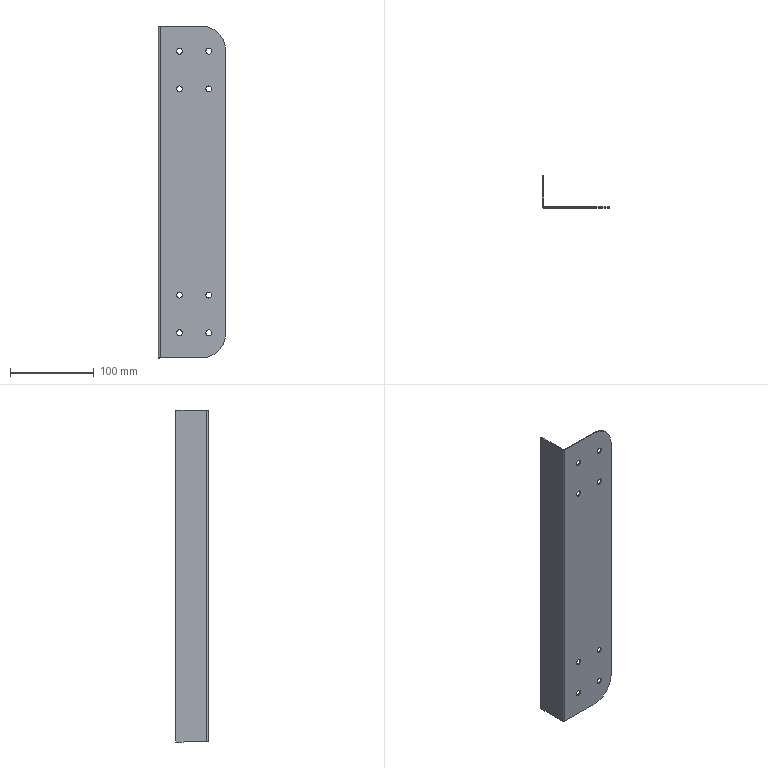Component | SolidWorks | dbj3-1_w13-1 | 1 solid | 32 faces | box 80 x 38.5 x 396 mm | volume 68176 mm3 | cylinder 20 | plane 12 | commonest cylinder face diameters 7 x16 58 x2 4 x1 1 x1
STEP:
#1=COLOUR_RGB('',0.7922,0.8196,0.9333);
#2=FILL_AREA_STYLE_COLOUR('',#1);
#3=FILL_AREA_STYLE('',(#2));
#4=SURFACE_STYLE_FILL_AREA(#3);
#5=SURFACE_SIDE_STYLE('',(#4));
#6=SURFACE_STYLE_USAGE(.BOTH.,#5);
#7=PRESENTATION_STYLE_ASSIGNMENT((#6));
#8=CARTESIAN_POINT('',(8.996,-31.014,8.445));
#9=VERTEX_POINT('',#8);
#10=CARTESIAN_POINT('',(8.996,-31.014,8.72));
#11=VERTEX_POINT('',#10);
#12=CARTESIAN_POINT('',(8.996,-31.014,8.583));
#13=DIRECTION('',(0.,-1.,0.));
#14=DIRECTION('',(0.,0.,1.));
#15=AXIS2_PLACEMENT_3D('',#12,#13,#14);
#16=CIRCLE('',#15,0.1378);
#17=EDGE_CURVE('',#9,#11,#16,.T.);
#18=ORIENTED_EDGE('',*,*,#17,.F.);
#19=CARTESIAN_POINT('',(8.996,-31.073,8.445));
#20=VERTEX_POINT('',#19);
#21=CARTESIAN_POINT('',(8.996,-30.679,8.445));
#22=DIRECTION('',(0.,-1.,0.));
#23=VECTOR('',#22,39.37);
#24=LINE('',#21,#23);
#25=EDGE_CURVE('',#9,#20,#24,.T.);
#26=ORIENTED_EDGE('',*,*,#25,.T.);
#27=CARTESIAN_POINT('',(8.996,-31.073,8.72));
#28=VERTEX_POINT('',#27);
#29=CARTESIAN_POINT('',(8.996,-31.073,8.583));
#30=DIRECTION('',(0.,-1.,0.));
#31=DIRECTION('',(0.,0.,-1.));
#32=AXIS2_PLACEMENT_3D('',#29,#30,#31);
#33=CIRCLE('',#32,0.1378);
#34=EDGE_CURVE('',#20,#28,#33,.T.);
#35=ORIENTED_EDGE('',*,*,#34,.T.);
#36=CARTESIAN_POINT('',(8.996,-30.679,8.72));
#37=DIRECTION('',(0.,-1.,0.));
#38=VECTOR('',#37,39.37);
#39=LINE('',#36,#38);
#40=EDGE_CURVE('',#11,#28,#39,.T.);
#41=ORIENTED_EDGE('',*,*,#40,.F.);
#42=EDGE_LOOP('',(#18,#26,#35,#41));
#43=FACE_OUTER_BOUND('',#42,.T.);
#44=CARTESIAN_POINT('',(8.996,-30.679,8.583));
#45=DIRECTION('',(0.,-1.,0.));
#46=DIRECTION('',(0.,0.,1.));
#47=AXIS2_PLACEMENT_3D('',#44,#45,#46);
#48=CYLINDRICAL_SURFACE('',#47,0.1378);
#49=ADVANCED_FACE('',(#43),#48,.F.);
#50=CARTESIAN_POINT('',(7.618,-31.014,8.445));
#51=VERTEX_POINT('',#50);
#52=CARTESIAN_POINT('',(7.618,-31.014,8.72));
#53=VERTEX_POINT('',#52);
#54=CARTESIAN_POINT('',(7.618,-31.014,8.583));
#55=DIRECTION('',(0.,-1.,0.));
#56=DIRECTION('',(0.,0.,1.));
#57=AXIS2_PLACEMENT_3D('',#54,#55,#56);
#58=CIRCLE('',#57,0.1378);
#59=EDGE_CURVE('',#51,#53,#58,.T.);
#60=ORIENTED_EDGE('',*,*,#59,.F.);
#61=CARTESIAN_POINT('',(7.618,-31.073,8.445));
#62=VERTEX_POINT('',#61);
#63=CARTESIAN_POINT('',(7.618,-30.679,8.445));
#64=DIRECTION('',(0.,-1.,0.));
#65=VECTOR('',#64,39.37);
#66=LINE('',#63,#65);
#67=EDGE_CURVE('',#51,#62,#66,.T.);
#68=ORIENTED_EDGE('',*,*,#67,.T.);
#69=CARTESIAN_POINT('',(7.618,-31.073,8.72));
#70=VERTEX_POINT('',#69);
#71=CARTESIAN_POINT('',(7.618,-31.073,8.583));
#72=DIRECTION('',(0.,-1.,0.));
#73=DIRECTION('',(0.,0.,-1.));
#74=AXIS2_PLACEMENT_3D('',#71,#72,#73);
#75=CIRCLE('',#74,0.1378);
#76=EDGE_CURVE('',#62,#70,#75,.T.);
#77=ORIENTED_EDGE('',*,*,#76,.T.);
#78=CARTESIAN_POINT('',(7.618,-30.679,8.72));
#79=DIRECTION('',(0.,-1.,0.));
#80=VECTOR('',#79,39.37);
#81=LINE('',#78,#80);
#82=EDGE_CURVE('',#53,#70,#81,.T.);
#83=ORIENTED_EDGE('',*,*,#82,.F.);
#84=EDGE_LOOP('',(#60,#68,#77,#83));
#85=FACE_OUTER_BOUND('',#84,.T.);
#86=CARTESIAN_POINT('',(7.618,-30.679,8.583));
#87=DIRECTION('',(0.,-1.,0.));
#88=DIRECTION('',(0.,0.,1.));
#89=AXIS2_PLACEMENT_3D('',#86,#87,#88);
#90=CYLINDRICAL_SURFACE('',#89,0.1378);
#91=ADVANCED_FACE('',(#85),#90,.F.);
#92=CARTESIAN_POINT('',(7.618,-31.014,6.673));
#93=VERTEX_POINT('',#92);
#94=CARTESIAN_POINT('',(7.618,-31.014,6.949));
#95=VERTEX_POINT('',#94);
#96=CARTESIAN_POINT('',(7.618,-31.014,6.811));
#97=DIRECTION('',(0.,-1.,0.));
#98=DIRECTION('',(0.,0.,1.));
#99=AXIS2_PLACEMENT_3D('',#96,#97,#98);
#100=CIRCLE('',#99,0.1378);
#101=EDGE_CURVE('',#93,#95,#100,.T.);
#102=ORIENTED_EDGE('',*,*,#101,.F.);
#103=CARTESIAN_POINT('',(7.618,-31.073,6.673));
#104=VERTEX_POINT('',#103);
#105=CARTESIAN_POINT('',(7.618,-30.679,6.673));
#106=DIRECTION('',(0.,-1.,0.));
#107=VECTOR('',#106,39.37);
#108=LINE('',#105,#107);
#109=EDGE_CURVE('',#93,#104,#108,.T.);
#110=ORIENTED_EDGE('',*,*,#109,.T.);
#111=CARTESIAN_POINT('',(7.618,-31.073,6.949));
#112=VERTEX_POINT('',#111);
#113=CARTESIAN_POINT('',(7.618,-31.073,6.811));
#114=DIRECTION('',(0.,-1.,0.));
#115=DIRECTION('',(0.,0.,-1.));
#116=AXIS2_PLACEMENT_3D('',#113,#114,#115);
#117=CIRCLE('',#116,0.1378);
#118=EDGE_CURVE('',#104,#112,#117,.T.);
#119=ORIENTED_EDGE('',*,*,#118,.T.);
#120=CARTESIAN_POINT('',(7.618,-30.679,6.949));
#121=DIRECTION('',(0.,-1.,0.));
#122=VECTOR('',#121,39.37);
#123=LINE('',#120,#122);
#124=EDGE_CURVE('',#95,#112,#123,.T.);
#125=ORIENTED_EDGE('',*,*,#124,.F.);
#126=EDGE_LOOP('',(#102,#110,#119,#125));
#127=FACE_OUTER_BOUND('',#126,.T.);
#128=CARTESIAN_POINT('',(7.618,-30.679,6.811));
#129=DIRECTION('',(0.,-1.,0.));
#130=DIRECTION('',(0.,0.,1.));
#131=AXIS2_PLACEMENT_3D('',#128,#129,#130);
#132=CYLINDRICAL_SURFACE('',#131,0.1378);
#133=ADVANCED_FACE('',(#127),#132,.F.);
#134=CARTESIAN_POINT('',(8.996,-31.014,6.673));
#135=VERTEX_POINT('',#134);
#136=CARTESIAN_POINT('',(8.996,-31.014,6.949));
#137=VERTEX_POINT('',#136);
#138=CARTESIAN_POINT('',(8.996,-31.014,6.811));
#139=DIRECTION('',(0.,-1.,0.));
#140=DIRECTION('',(0.,0.,1.));
#141=AXIS2_PLACEMENT_3D('',#138,#139,#140);
#142=CIRCLE('',#141,0.1378);
#143=EDGE_CURVE('',#135,#137,#142,.T.);
#144=ORIENTED_EDGE('',*,*,#143,.F.);
#145=CARTESIAN_POINT('',(8.996,-31.073,6.673));
#146=VERTEX_POINT('',#145);
#147=CARTESIAN_POINT('',(8.996,-30.679,6.673));
#148=DIRECTION('',(0.,-1.,0.));
#149=VECTOR('',#148,39.37);
#150=LINE('',#147,#149);
#151=EDGE_CURVE('',#135,#146,#150,.T.);
#152=ORIENTED_EDGE('',*,*,#151,.T.);
#153=CARTESIAN_POINT('',(8.996,-31.073,6.949));
#154=VERTEX_POINT('',#153);
#155=CARTESIAN_POINT('',(8.996,-31.073,6.811));
#156=DIRECTION('',(0.,-1.,0.));
#157=DIRECTION('',(0.,0.,-1.));
#158=AXIS2_PLACEMENT_3D('',#155,#156,#157);
#159=CIRCLE('',#158,0.1378);
#160=EDGE_CURVE('',#146,#154,#159,.T.);
#161=ORIENTED_EDGE('',*,*,#160,.T.);
#162=CARTESIAN_POINT('',(8.996,-30.679,6.949));
#163=DIRECTION('',(0.,-1.,0.));
#164=VECTOR('',#163,39.37);
#165=LINE('',#162,#164);
#166=EDGE_CURVE('',#137,#154,#165,.T.);
#167=ORIENTED_EDGE('',*,*,#166,.F.);
#168=EDGE_LOOP('',(#144,#152,#161,#167));
#169=FACE_OUTER_BOUND('',#168,.T.);
#170=CARTESIAN_POINT('',(8.996,-30.679,6.811));
#171=DIRECTION('',(0.,-1.,0.));
#172=DIRECTION('',(0.,0.,1.));
#173=AXIS2_PLACEMENT_3D('',#170,#171,#172);
#174=CYLINDRICAL_SURFACE('',#173,0.1378);
#175=ADVANCED_FACE('',(#169),#174,.F.);
#176=CARTESIAN_POINT('',(8.996,-31.014,-3.012));
#177=VERTEX_POINT('',#176);
#178=CARTESIAN_POINT('',(8.996,-31.014,-2.736));
#179=VERTEX_POINT('',#178);
#180=CARTESIAN_POINT('',(8.996,-31.014,-2.874));
#181=DIRECTION('',(0.,-1.,0.));
#182=DIRECTION('',(0.,0.,1.));
#183=AXIS2_PLACEMENT_3D('',#180,#181,#182);
#184=CIRCLE('',#183,0.1378);
#185=EDGE_CURVE('',#177,#179,#184,.T.);
#186=ORIENTED_EDGE('',*,*,#185,.F.);
#187=CARTESIAN_POINT('',(8.996,-31.073,-3.012));
#188=VERTEX_POINT('',#187);
#189=CARTESIAN_POINT('',(8.996,-30.679,-3.012));
#190=DIRECTION('',(0.,-1.,0.));
#191=VECTOR('',#190,39.37);
#192=LINE('',#189,#191);
#193=EDGE_CURVE('',#177,#188,#192,.T.);
#194=ORIENTED_EDGE('',*,*,#193,.T.);
#195=CARTESIAN_POINT('',(8.996,-31.073,-2.736));
#196=VERTEX_POINT('',#195);
#197=CARTESIAN_POINT('',(8.996,-31.073,-2.874));
#198=DIRECTION('',(0.,-1.,0.));
#199=DIRECTION('',(0.,0.,1.));
#200=AXIS2_PLACEMENT_3D('',#197,#198,#199);
#201=CIRCLE('',#200,0.1378);
#202=EDGE_CURVE('',#188,#196,#201,.T.);
#203=ORIENTED_EDGE('',*,*,#202,.T.);
#204=CARTESIAN_POINT('',(8.996,-30.679,-2.736));
#205=DIRECTION('',(0.,-1.,0.));
#206=VECTOR('',#205,39.37);
#207=LINE('',#204,#206);
#208=EDGE_CURVE('',#179,#196,#207,.T.);
#209=ORIENTED_EDGE('',*,*,#208,.F.);
#210=EDGE_LOOP('',(#186,#194,#203,#209));
#211=FACE_OUTER_BOUND('',#210,.T.);
#212=CARTESIAN_POINT('',(8.996,-30.679,-2.874));
#213=DIRECTION('',(0.,-1.,0.));
#214=DIRECTION('',(0.,0.,1.));
#215=AXIS2_PLACEMENT_3D('',#212,#213,#214);
#216=CYLINDRICAL_SURFACE('',#215,0.1378);
#217=ADVANCED_FACE('',(#211),#216,.F.);
#218=CARTESIAN_POINT('',(7.618,-31.014,-3.012));
#219=VERTEX_POINT('',#218);
#220=CARTESIAN_POINT('',(7.618,-31.014,-2.736));
#221=VERTEX_POINT('',#220);
#222=CARTESIAN_POINT('',(7.618,-31.014,-2.874));
#223=DIRECTION('',(0.,-1.,0.));
#224=DIRECTION('',(0.,0.,1.));
#225=AXIS2_PLACEMENT_3D('',#222,#223,#224);
#226=CIRCLE('',#225,0.1378);
#227=EDGE_CURVE('',#219,#221,#226,.T.);
#228=ORIENTED_EDGE('',*,*,#227,.F.);
#229=CARTESIAN_POINT('',(7.618,-31.073,-3.012));
#230=VERTEX_POINT('',#229);
#231=CARTESIAN_POINT('',(7.618,-30.679,-3.012));
#232=DIRECTION('',(0.,-1.,0.));
#233=VECTOR('',#232,39.37);
#234=LINE('',#231,#233);
#235=EDGE_CURVE('',#219,#230,#234,.T.);
#236=ORIENTED_EDGE('',*,*,#235,.T.);
#237=CARTESIAN_POINT('',(7.618,-31.073,-2.736));
#238=VERTEX_POINT('',#237);
#239=CARTESIAN_POINT('',(7.618,-31.073,-2.874));
#240=DIRECTION('',(0.,-1.,0.));
#241=DIRECTION('',(0.,0.,1.));
#242=AXIS2_PLACEMENT_3D('',#239,#240,#241);
#243=CIRCLE('',#242,0.1378);
#244=EDGE_CURVE('',#230,#238,#243,.T.);
#245=ORIENTED_EDGE('',*,*,#244,.T.);
#246=CARTESIAN_POINT('',(7.618,-30.679,-2.736));
#247=DIRECTION('',(0.,-1.,0.));
#248=VECTOR('',#247,39.37);
#249=LINE('',#246,#248);
#250=EDGE_CURVE('',#221,#238,#249,.T.);
#251=ORIENTED_EDGE('',*,*,#250,.F.);
#252=EDGE_LOOP('',(#228,#236,#245,#251));
#253=FACE_OUTER_BOUND('',#252,.T.);
#254=CARTESIAN_POINT('',(7.618,-30.679,-2.874));
#255=DIRECTION('',(0.,-1.,0.));
#256=DIRECTION('',(0.,0.,1.));
#257=AXIS2_PLACEMENT_3D('',#254,#255,#256);
#258=CYLINDRICAL_SURFACE('',#257,0.1378);
#259=ADVANCED_FACE('',(#253),#258,.F.);
#260=CARTESIAN_POINT('',(7.618,-31.014,-4.783));
#261=VERTEX_POINT('',#260);
#262=CARTESIAN_POINT('',(7.618,-31.014,-4.508));
#263=VERTEX_POINT('',#262);
#264=CARTESIAN_POINT('',(7.618,-31.014,-4.646));
#265=DIRECTION('',(0.,-1.,0.));
#266=DIRECTION('',(0.,0.,1.));
#267=AXIS2_PLACEMENT_3D('',#264,#265,#266);
#268=CIRCLE('',#267,0.1378);
#269=EDGE_CURVE('',#261,#263,#268,.T.);
#270=ORIENTED_EDGE('',*,*,#269,.F.);
#271=CARTESIAN_POINT('',(7.618,-31.073,-4.783));
#272=VERTEX_POINT('',#271);
#273=CARTESIAN_POINT('',(7.618,-30.679,-4.783));
#274=DIRECTION('',(0.,-1.,0.));
#275=VECTOR('',#274,39.37);
#276=LINE('',#273,#275);
#277=EDGE_CURVE('',#261,#272,#276,.T.);
#278=ORIENTED_EDGE('',*,*,#277,.T.);
#279=CARTESIAN_POINT('',(7.618,-31.073,-4.508));
#280=VERTEX_POINT('',#279);
#281=CARTESIAN_POINT('',(7.618,-31.073,-4.646));
#282=DIRECTION('',(0.,-1.,0.));
#283=DIRECTION('',(0.,0.,1.));
#284=AXIS2_PLACEMENT_3D('',#281,#282,#283);
#285=CIRCLE('',#284,0.1378);
#286=EDGE_CURVE('',#272,#280,#285,.T.);
#287=ORIENTED_EDGE('',*,*,#286,.T.);
#288=CARTESIAN_POINT('',(7.618,-30.679,-4.508));
#289=DIRECTION('',(0.,-1.,0.));
#290=VECTOR('',#289,39.37);
#291=LINE('',#288,#290);
#292=EDGE_CURVE('',#263,#280,#291,.T.);
#293=ORIENTED_EDGE('',*,*,#292,.F.);
#294=EDGE_LOOP('',(#270,#278,#287,#293));
#295=FACE_OUTER_BOUND('',#294,.T.);
#296=CARTESIAN_POINT('',(7.618,-30.679,-4.646));
#297=DIRECTION('',(0.,-1.,0.));
#298=DIRECTION('',(0.,0.,1.));
#299=AXIS2_PLACEMENT_3D('',#296,#297,#298);
#300=CYLINDRICAL_SURFACE('',#299,0.1378);
#301=ADVANCED_FACE('',(#295),#300,.F.);
#302=CARTESIAN_POINT('',(8.996,-31.014,-4.783));
#303=VERTEX_POINT('',#302);
#304=CARTESIAN_POINT('',(8.996,-31.014,-4.508));
#305=VERTEX_POINT('',#304);
#306=CARTESIAN_POINT('',(8.996,-31.014,-4.646));
#307=DIRECTION('',(0.,-1.,0.));
#308=DIRECTION('',(0.,0.,1.));
#309=AXIS2_PLACEMENT_3D('',#306,#307,#308);
#310=CIRCLE('',#309,0.1378);
#311=EDGE_CURVE('',#303,#305,#310,.T.);
#312=ORIENTED_EDGE('',*,*,#311,.F.);
#313=CARTESIAN_POINT('',(8.996,-31.073,-4.783));
#314=VERTEX_POINT('',#313);
#315=CARTESIAN_POINT('',(8.996,-30.679,-4.783));
#316=DIRECTION('',(0.,-1.,0.));
#317=VECTOR('',#316,39.37);
#318=LINE('',#315,#317);
#319=EDGE_CURVE('',#303,#314,#318,.T.);
#320=ORIENTED_EDGE('',*,*,#319,.T.);
#321=CARTESIAN_POINT('',(8.996,-31.073,-4.508));
#322=VERTEX_POINT('',#321);
#323=CARTESIAN_POINT('',(8.996,-31.073,-4.646));
#324=DIRECTION('',(0.,-1.,0.));
#325=DIRECTION('',(0.,0.,1.));
#326=AXIS2_PLACEMENT_3D('',#323,#324,#325);
#327=CIRCLE('',#326,0.1378);
#328=EDGE_CURVE('',#314,#322,#327,.T.);
#329=ORIENTED_EDGE('',*,*,#328,.T.);
#330=CARTESIAN_POINT('',(8.996,-30.679,-4.508));
#331=DIRECTION('',(0.,-1.,0.));
#332=VECTOR('',#331,39.37);
#333=LINE('',#330,#332);
#334=EDGE_CURVE('',#305,#322,#333,.T.);
#335=ORIENTED_EDGE('',*,*,#334,.F.);
#336=EDGE_LOOP('',(#312,#320,#329,#335));
#337=FACE_OUTER_BOUND('',#336,.T.);
#338=CARTESIAN_POINT('',(8.996,-30.679,-4.646));
#339=DIRECTION('',(0.,-1.,0.));
#340=DIRECTION('',(0.,0.,1.));
#341=AXIS2_PLACEMENT_3D('',#338,#339,#340);
#342=CYLINDRICAL_SURFACE('',#341,0.1378);
#343=ADVANCED_FACE('',(#337),#342,.F.);
#344=CARTESIAN_POINT('',(6.634,-30.994,9.764));
#345=VERTEX_POINT('',#344);
#346=CARTESIAN_POINT('',(6.693,-30.994,9.764));
#347=VERTEX_POINT('',#346);
#348=CARTESIAN_POINT('',(6.634,-30.994,9.764));
#349=DIRECTION('',(1.,0.,-0.));
#350=VECTOR('',#349,39.37);
#351=LINE('',#348,#350);
#352=EDGE_CURVE('',#345,#347,#351,.T.);
#353=ORIENTED_EDGE('',*,*,#352,.F.);
#354=CARTESIAN_POINT('',(6.713,-31.073,9.764));
#355=VERTEX_POINT('',#354);
#356=CARTESIAN_POINT('',(6.713,-30.994,9.764));
#357=DIRECTION('',(-0.,-0.,-1.));
#358=DIRECTION('',(-1.,0.,0.));
#359=AXIS2_PLACEMENT_3D('',#356,#357,#358);
#360=CIRCLE('',#359,0.07874);
#361=EDGE_CURVE('',#355,#345,#360,.T.);
#362=ORIENTED_EDGE('',*,*,#361,.F.);
#363=CARTESIAN_POINT('',(6.713,-31.014,9.764));
#364=VERTEX_POINT('',#363);
#365=CARTESIAN_POINT('',(6.713,-31.014,9.764));
#366=DIRECTION('',(0.,-1.,0.));
#367=VECTOR('',#366,39.37);
#368=LINE('',#365,#367);
#369=EDGE_CURVE('',#364,#355,#368,.T.);
#370=ORIENTED_EDGE('',*,*,#369,.F.);
#371=CARTESIAN_POINT('',(6.713,-30.994,9.764));
#372=DIRECTION('',(-0.,-0.,-1.));
#373=DIRECTION('',(-1.,0.,0.));
#374=AXIS2_PLACEMENT_3D('',#371,#372,#373);
#375=CIRCLE('',#374,0.01969);
#376=EDGE_CURVE('',#364,#347,#375,.T.);
#377=ORIENTED_EDGE('',*,*,#376,.T.);
#378=EDGE_LOOP('',(#353,#362,#370,#377));
#379=FACE_OUTER_BOUND('',#378,.T.);
#380=CARTESIAN_POINT('',(6.634,-30.994,9.764));
#381=DIRECTION('',(0.,0.,1.));
#382=DIRECTION('',(-1.,-0.,0.));
#383=AXIS2_PLACEMENT_3D('',#380,#381,#382);
#384=PLANE('',#383);
#385=ADVANCED_FACE('',(#379),#384,.T.);
#386=CARTESIAN_POINT('',(6.634,-29.557,9.764));
#387=VERTEX_POINT('',#386);
#388=CARTESIAN_POINT('',(6.634,-31.073,9.764));
#389=DIRECTION('',(-0.,1.,-0.));
#390=VECTOR('',#389,39.37);
#391=LINE('',#388,#390);
#392=EDGE_CURVE('',#345,#387,#391,.T.);
#393=ORIENTED_EDGE('',*,*,#392,.F.);
#394=ORIENTED_EDGE('',*,*,#352,.T.);
#395=CARTESIAN_POINT('',(6.693,-29.557,9.764));
#396=VERTEX_POINT('',#395);
#397=CARTESIAN_POINT('',(6.693,-31.073,9.764));
#398=DIRECTION('',(-0.,1.,-0.));
#399=VECTOR('',#398,39.37);
#400=LINE('',#397,#399);
#401=EDGE_CURVE('',#347,#396,#400,.T.);
#402=ORIENTED_EDGE('',*,*,#401,.T.);
#403=CARTESIAN_POINT('',(6.634,-29.557,9.764));
#404=DIRECTION('',(1.,0.,-0.));
#405=VECTOR('',#404,39.37);
#406=LINE('',#403,#405);
#407=EDGE_CURVE('',#387,#396,#406,.T.);
#408=ORIENTED_EDGE('',*,*,#407,.F.);
#409=EDGE_LOOP('',(#393,#394,#402,#408));
#410=FACE_OUTER_BOUND('',#409,.T.);
#411=CARTESIAN_POINT('',(6.713,-31.014,9.764));
#412=DIRECTION('',(0.,0.,1.));
#413=DIRECTION('',(-1.,-0.,0.));
#414=AXIS2_PLACEMENT_3D('',#411,#412,#413);
#415=PLANE('',#414);
#416=ADVANCED_FACE('',(#410),#415,.T.);
#417=CARTESIAN_POINT('',(6.713,-31.073,-5.827));
#418=VERTEX_POINT('',#417);
#419=CARTESIAN_POINT('',(6.713,-31.014,-5.827));
#420=VERTEX_POINT('',#419);
#421=CARTESIAN_POINT('',(6.713,-31.073,-5.827));
#422=DIRECTION('',(-0.,1.,-0.));
#423=VECTOR('',#422,39.37);
#424=LINE('',#421,#423);
#425=EDGE_CURVE('',#418,#420,#424,.T.);
#426=ORIENTED_EDGE('',*,*,#425,.F.);
#427=CARTESIAN_POINT('',(6.634,-30.994,-5.827));
#428=VERTEX_POINT('',#427);
#429=CARTESIAN_POINT('',(6.713,-30.994,-5.827));
#430=DIRECTION('',(-0.,-0.,-1.));
#431=DIRECTION('',(-1.,0.,0.));
#432=AXIS2_PLACEMENT_3D('',#429,#430,#431);
#433=CIRCLE('',#432,0.07874);
#434=EDGE_CURVE('',#418,#428,#433,.T.);
#435=ORIENTED_EDGE('',*,*,#434,.T.);
#436=CARTESIAN_POINT('',(6.693,-30.994,-5.827));
#437=VERTEX_POINT('',#436);
#438=CARTESIAN_POINT('',(6.693,-30.994,-5.827));
#439=DIRECTION('',(-1.,-0.,0.));
#440=VECTOR('',#439,39.37);
#441=LINE('',#438,#440);
#442=EDGE_CURVE('',#437,#428,#441,.T.);
#443=ORIENTED_EDGE('',*,*,#442,.F.);
#444=CARTESIAN_POINT('',(6.713,-30.994,-5.827));
#445=DIRECTION('',(-0.,-0.,-1.));
#446=DIRECTION('',(-1.,0.,0.));
#447=AXIS2_PLACEMENT_3D('',#444,#445,#446);
#448=CIRCLE('',#447,0.01969);
#449=EDGE_CURVE('',#420,#437,#448,.T.);
#450=ORIENTED_EDGE('',*,*,#449,.F.);
#451=EDGE_LOOP('',(#426,#435,#443,#450));
#452=FACE_OUTER_BOUND('',#451,.T.);
#453=CARTESIAN_POINT('',(6.713,-31.073,-5.827));
#454=DIRECTION('',(-0.,-0.,-1.));
#455=DIRECTION('',(1.,0.,-0.));
#456=AXIS2_PLACEMENT_3D('',#453,#454,#455);
#457=PLANE('',#456);
#458=ADVANCED_FACE('',(#452),#457,.T.);
#459=CARTESIAN_POINT('',(8.642,-31.014,-5.827));
#460=VERTEX_POINT('',#459);
#461=CARTESIAN_POINT('',(9.783,-31.014,-5.827));
#462=DIRECTION('',(-1.,-0.,0.));
#463=VECTOR('',#462,39.37);
#464=LINE('',#461,#463);
#465=EDGE_CURVE('',#460,#420,#464,.T.);
#466=ORIENTED_EDGE('',*,*,#465,.F.);
#467=CARTESIAN_POINT('',(8.642,-31.073,-5.827));
#468=VERTEX_POINT('',#467);
#469=CARTESIAN_POINT('',(8.642,-30.994,-5.827));
#470=DIRECTION('',(0.,-1.,0.));
#471=VECTOR('',#470,39.37);
#472=LINE('',#469,#471);
#473=EDGE_CURVE('',#460,#468,#472,.T.);
#474=ORIENTED_EDGE('',*,*,#473,.T.);
#475=CARTESIAN_POINT('',(9.783,-31.073,-5.827));
#476=DIRECTION('',(-1.,-0.,0.));
#477=VECTOR('',#476,39.37);
#478=LINE('',#475,#477);
#479=EDGE_CURVE('',#468,#418,#478,.T.);
#480=ORIENTED_EDGE('',*,*,#479,.T.);
#481=ORIENTED_EDGE('',*,*,#425,.T.);
#482=EDGE_LOOP('',(#466,#474,#480,#481));
#483=FACE_OUTER_BOUND('',#482,.T.);
#484=CARTESIAN_POINT('',(6.693,-30.994,-5.827));
#485=DIRECTION('',(-0.,-0.,-1.));
#486=DIRECTION('',(1.,0.,-0.));
#487=AXIS2_PLACEMENT_3D('',#484,#485,#486);
#488=PLANE('',#487);
#489=ADVANCED_FACE('',(#483),#488,.T.);
#490=CARTESIAN_POINT('',(6.693,-29.557,-5.827));
#491=VERTEX_POINT('',#490);
#492=CARTESIAN_POINT('',(6.693,-31.073,-5.827));
#493=DIRECTION('',(-0.,1.,-0.));
#494=VECTOR('',#493,39.37);
#495=LINE('',#492,#494);
#496=EDGE_CURVE('',#437,#491,#495,.T.);
#497=ORIENTED_EDGE('',*,*,#496,.T.);
#498=CARTESIAN_POINT('',(6.693,-29.557,9.764));
#499=DIRECTION('',(-0.,-0.,-1.));
#500=VECTOR('',#499,39.37);
#501=LINE('',#498,#500);
#502=EDGE_CURVE('',#396,#491,#501,.T.);
#503=ORIENTED_EDGE('',*,*,#502,.F.);
#504=ORIENTED_EDGE('',*,*,#401,.F.);
#505=CARTESIAN_POINT('',(6.693,-30.994,9.764));
#506=DIRECTION('',(-0.,-0.,-1.));
#507=VECTOR('',#506,39.37);
#508=LINE('',#505,#507);
#509=EDGE_CURVE('',#347,#437,#508,.T.);
#510=ORIENTED_EDGE('',*,*,#509,.T.);
#511=EDGE_LOOP('',(#497,#503,#504,#510));
#512=FACE_OUTER_BOUND('',#511,.T.);
#513=CARTESIAN_POINT('',(6.693,-31.073,9.764));
#514=DIRECTION('',(-1.,-0.,0.));
#515=DIRECTION('',(0.,-1.,0.));
#516=AXIS2_PLACEMENT_3D('',#513,#514,#515);
#517=PLANE('',#516);
#518=ADVANCED_FACE('',(#512),#517,.F.);
#519=CARTESIAN_POINT('',(6.634,-29.557,-5.827));
#520=VERTEX_POINT('',#519);
#521=CARTESIAN_POINT('',(6.634,-29.557,-5.827));
#522=DIRECTION('',(1.,0.,-0.));
#523=VECTOR('',#522,39.37);
#524=LINE('',#521,#523);
#525=EDGE_CURVE('',#520,#491,#524,.T.);
#526=ORIENTED_EDGE('',*,*,#525,.F.);
#527=CARTESIAN_POINT('',(6.634,-29.557,9.764));
#528=DIRECTION('',(-0.,-0.,-1.));
#529=VECTOR('',#528,39.37);
#530=LINE('',#527,#529);
#531=EDGE_CURVE('',#387,#520,#530,.T.);
#532=ORIENTED_EDGE('',*,*,#531,.F.);
#533=ORIENTED_EDGE('',*,*,#407,.T.);
#534=ORIENTED_EDGE('',*,*,#502,.T.);
#535=EDGE_LOOP('',(#526,#532,#533,#534));
#536=FACE_OUTER_BOUND('',#535,.T.);
#537=CARTESIAN_POINT('',(6.634,-29.557,9.764));
#538=DIRECTION('',(-0.,1.,-0.));
#539=DIRECTION('',(-0.,-0.,-1.));
#540=AXIS2_PLACEMENT_3D('',#537,#538,#539);
#541=PLANE('',#540);
#542=ADVANCED_FACE('',(#536),#541,.T.);
#543=CARTESIAN_POINT('',(6.634,-31.073,-5.827));
#544=DIRECTION('',(-0.,1.,-0.));
#545=VECTOR('',#544,39.37);
#546=LINE('',#543,#545);
#547=EDGE_CURVE('',#428,#520,#546,.T.);
#548=ORIENTED_EDGE('',*,*,#547,.F.);
#549=CARTESIAN_POINT('',(6.634,-30.994,9.764));
#550=DIRECTION('',(-0.,-0.,-1.));
#551=VECTOR('',#550,39.37);
#552=LINE('',#549,#551);
#553=EDGE_CURVE('',#345,#428,#552,.T.);
#554=ORIENTED_EDGE('',*,*,#553,.F.);
#555=ORIENTED_EDGE('',*,*,#392,.T.);
#556=ORIENTED_EDGE('',*,*,#531,.T.);
#557=EDGE_LOOP('',(#548,#554,#555,#556));
#558=FACE_OUTER_BOUND('',#557,.T.);
#559=CARTESIAN_POINT('',(6.634,-31.073,9.764));
#560=DIRECTION('',(-1.,-0.,0.));
#561=DIRECTION('',(0.,-1.,0.));
#562=AXIS2_PLACEMENT_3D('',#559,#560,#561);
#563=PLANE('',#562);
#564=ADVANCED_FACE('',(#558),#563,.T.);
#565=ORIENTED_EDGE('',*,*,#434,.F.);
#566=CARTESIAN_POINT('',(6.713,-31.073,9.764));
#567=DIRECTION('',(-0.,-0.,-1.));
#568=VECTOR('',#567,39.37);
#569=LINE('',#566,#568);
#570=EDGE_CURVE('',#355,#418,#569,.T.);
#571=ORIENTED_EDGE('',*,*,#570,.F.);
#572=ORIENTED_EDGE('',*,*,#361,.T.);
#573=ORIENTED_EDGE('',*,*,#553,.T.);
#574=EDGE_LOOP('',(#565,#571,#572,#573));
#575=FACE_OUTER_BOUND('',#574,.T.);
#576=CARTESIAN_POINT('',(6.713,-30.994,9.764));
#577=DIRECTION('',(-0.,-0.,-1.));
#578=DIRECTION('',(1.,0.,0.));
#579=AXIS2_PLACEMENT_3D('',#576,#577,#578);
#580=CYLINDRICAL_SURFACE('',#579,0.07874);
#581=ADVANCED_FACE('',(#575),#580,.T.);
#582=CARTESIAN_POINT('',(8.996,-31.073,8.583));
#583=DIRECTION('',(0.,-1.,0.));
#584=DIRECTION('',(0.,0.,-1.));
#585=AXIS2_PLACEMENT_3D('',#582,#583,#584);
#586=CIRCLE('',#585,0.1378);
#587=EDGE_CURVE('',#28,#20,#586,.T.);
#588=ORIENTED_EDGE('',*,*,#587,.F.);
#589=ORIENTED_EDGE('',*,*,#34,.F.);
#590=EDGE_LOOP('',(#588,#589));
#591=FACE_BOUND('',#590,.T.);
#592=CARTESIAN_POINT('',(7.618,-31.073,8.583));
#593=DIRECTION('',(0.,-1.,0.));
#594=DIRECTION('',(0.,0.,-1.));
#595=AXIS2_PLACEMENT_3D('',#592,#593,#594);
#596=CIRCLE('',#595,0.1378);
#597=EDGE_CURVE('',#70,#62,#596,.T.);
#598=ORIENTED_EDGE('',*,*,#597,.F.);
#599=ORIENTED_EDGE('',*,*,#76,.F.);
#600=EDGE_LOOP('',(#598,#599));
#601=FACE_BOUND('',#600,.T.);
#602=CARTESIAN_POINT('',(7.618,-31.073,6.811));
#603=DIRECTION('',(0.,-1.,0.));
#604=DIRECTION('',(0.,0.,-1.));
#605=AXIS2_PLACEMENT_3D('',#602,#603,#604);
#606=CIRCLE('',#605,0.1378);
#607=EDGE_CURVE('',#112,#104,#606,.T.);
#608=ORIENTED_EDGE('',*,*,#607,.F.);
#609=ORIENTED_EDGE('',*,*,#118,.F.);
#610=EDGE_LOOP('',(#608,#609));
#611=FACE_BOUND('',#610,.T.);
#612=CARTESIAN_POINT('',(8.996,-31.073,6.811));
#613=DIRECTION('',(0.,-1.,0.));
#614=DIRECTION('',(0.,0.,-1.));
#615=AXIS2_PLACEMENT_3D('',#612,#613,#614);
#616=CIRCLE('',#615,0.1378);
#617=EDGE_CURVE('',#154,#146,#616,.T.);
#618=ORIENTED_EDGE('',*,*,#617,.F.);
#619=ORIENTED_EDGE('',*,*,#160,.F.);
#620=EDGE_LOOP('',(#618,#619));
#621=FACE_BOUND('',#620,.T.);
#622=CARTESIAN_POINT('',(8.996,-31.073,-2.874));
#623=DIRECTION('',(0.,-1.,0.));
#624=DIRECTION('',(0.,0.,1.));
#625=AXIS2_PLACEMENT_3D('',#622,#623,#624);
#626=CIRCLE('',#625,0.1378);
#627=EDGE_CURVE('',#196,#188,#626,.T.);
#628=ORIENTED_EDGE('',*,*,#627,.F.);
#629=ORIENTED_EDGE('',*,*,#202,.F.);
#630=EDGE_LOOP('',(#628,#629));
#631=FACE_BOUND('',#630,.T.);
#632=CARTESIAN_POINT('',(7.618,-31.073,-2.874));
#633=DIRECTION('',(0.,-1.,0.));
#634=DIRECTION('',(0.,0.,1.));
#635=AXIS2_PLACEMENT_3D('',#632,#633,#634);
#636=CIRCLE('',#635,0.1378);
#637=EDGE_CURVE('',#238,#230,#636,.T.);
#638=ORIENTED_EDGE('',*,*,#637,.F.);
#639=ORIENTED_EDGE('',*,*,#244,.F.);
#640=EDGE_LOOP('',(#638,#639));
#641=FACE_BOUND('',#640,.T.);
#642=CARTESIAN_POINT('',(7.618,-31.073,-4.646));
#643=DIRECTION('',(0.,-1.,0.));
#644=DIRECTION('',(0.,0.,1.));
#645=AXIS2_PLACEMENT_3D('',#642,#643,#644);
#646=CIRCLE('',#645,0.1378);
#647=EDGE_CURVE('',#280,#272,#646,.T.);
#648=ORIENTED_EDGE('',*,*,#647,.F.);
#649=ORIENTED_EDGE('',*,*,#286,.F.);
#650=EDGE_LOOP('',(#648,#649));
#651=FACE_BOUND('',#650,.T.);
#652=CARTESIAN_POINT('',(8.996,-31.073,-4.646));
#653=DIRECTION('',(0.,-1.,0.));
#654=DIRECTION('',(0.,0.,1.));
#655=AXIS2_PLACEMENT_3D('',#652,#653,#654);
#656=CIRCLE('',#655,0.1378);
#657=EDGE_CURVE('',#322,#314,#656,.T.);
#658=ORIENTED_EDGE('',*,*,#657,.F.);
#659=ORIENTED_EDGE('',*,*,#328,.F.);
#660=EDGE_LOOP('',(#658,#659));
#661=FACE_BOUND('',#660,.T.);
#662=CARTESIAN_POINT('',(9.783,-31.073,8.622));
#663=VERTEX_POINT('',#662);
#664=CARTESIAN_POINT('',(9.783,-31.073,-4.685));
#665=VERTEX_POINT('',#664);
#666=CARTESIAN_POINT('',(9.783,-31.073,9.764));
#667=DIRECTION('',(-0.,-0.,-1.));
#668=VECTOR('',#667,39.37);
#669=LINE('',#666,#668);
#670=EDGE_CURVE('',#663,#665,#669,.T.);
#671=ORIENTED_EDGE('',*,*,#670,.F.);
#672=CARTESIAN_POINT('',(8.642,-31.073,9.764));
#673=VERTEX_POINT('',#672);
#674=CARTESIAN_POINT('',(8.642,-31.073,8.622));
#675=DIRECTION('',(0.,-1.,0.));
#676=DIRECTION('',(0.,0.,1.));
#677=AXIS2_PLACEMENT_3D('',#674,#675,#676);
#678=CIRCLE('',#677,1.142);
#679=EDGE_CURVE('',#663,#673,#678,.T.);
#680=ORIENTED_EDGE('',*,*,#679,.T.);
#681=CARTESIAN_POINT('',(9.783,-31.073,9.764));
#682=DIRECTION('',(-1.,-0.,0.));
#683=VECTOR('',#682,39.37);
#684=LINE('',#681,#683);
#685=EDGE_CURVE('',#673,#355,#684,.T.);
#686=ORIENTED_EDGE('',*,*,#685,.T.);
#687=ORIENTED_EDGE('',*,*,#570,.T.);
#688=ORIENTED_EDGE('',*,*,#479,.F.);
#689=CARTESIAN_POINT('',(8.642,-31.073,-4.685));
#690=DIRECTION('',(0.,-1.,0.));
#691=DIRECTION('',(0.,0.,1.));
#692=AXIS2_PLACEMENT_3D('',#689,#690,#691);
#693=CIRCLE('',#692,1.142);
#694=EDGE_CURVE('',#468,#665,#693,.T.);
#695=ORIENTED_EDGE('',*,*,#694,.T.);
#696=EDGE_LOOP('',(#671,#680,#686,#687,#688,#695));
#697=FACE_OUTER_BOUND('',#696,.T.);
#698=CARTESIAN_POINT('',(9.783,-31.073,9.764));
#699=DIRECTION('',(0.,-1.,0.));
#700=DIRECTION('',(0.,0.,1.));
#701=AXIS2_PLACEMENT_3D('',#698,#699,#700);
#702=PLANE('',#701);
#703=ADVANCED_FACE('',(#591,#601,#611,#621,#631,#641,#651,#661,#697),#702,.T.);
#704=CARTESIAN_POINT('',(9.783,-31.014,8.622));
#705=VERTEX_POINT('',#704);
#706=CARTESIAN_POINT('',(9.783,-31.014,-4.685));
#707=VERTEX_POINT('',#706);
#708=CARTESIAN_POINT('',(9.783,-31.014,9.764));
#709=DIRECTION('',(-0.,-0.,-1.));
#710=VECTOR('',#709,39.37);
#711=LINE('',#708,#710);
#712=EDGE_CURVE('',#705,#707,#711,.T.);
#713=ORIENTED_EDGE('',*,*,#712,.F.);
#714=CARTESIAN_POINT('',(9.783,-31.014,8.622));
#715=DIRECTION('',(0.,-1.,0.));
#716=VECTOR('',#715,39.37);
#717=LINE('',#714,#716);
#718=EDGE_CURVE('',#705,#663,#717,.T.);
#719=ORIENTED_EDGE('',*,*,#718,.T.);
#720=ORIENTED_EDGE('',*,*,#670,.T.);
#721=CARTESIAN_POINT('',(9.783,-31.014,-4.685));
#722=DIRECTION('',(-0.,1.,-0.));
#723=VECTOR('',#722,39.37);
#724=LINE('',#721,#723);
#725=EDGE_CURVE('',#665,#707,#724,.T.);
#726=ORIENTED_EDGE('',*,*,#725,.T.);
#727=EDGE_LOOP('',(#713,#719,#720,#726));
#728=FACE_OUTER_BOUND('',#727,.T.);
#729=CARTESIAN_POINT('',(9.783,-31.014,9.764));
#730=DIRECTION('',(1.,0.,-0.));
#731=DIRECTION('',(0.,0.,1.));
#732=AXIS2_PLACEMENT_3D('',#729,#730,#731);
#733=PLANE('',#732);
#734=ADVANCED_FACE('',(#728),#733,.T.);
#735=CARTESIAN_POINT('',(8.996,-31.014,8.583));
#736=DIRECTION('',(0.,-1.,0.));
#737=DIRECTION('',(0.,0.,1.));
#738=AXIS2_PLACEMENT_3D('',#735,#736,#737);
#739=CIRCLE('',#738,0.1378);
#740=EDGE_CURVE('',#11,#9,#739,.T.);
#741=ORIENTED_EDGE('',*,*,#740,.T.);
#742=ORIENTED_EDGE('',*,*,#17,.T.);
#743=EDGE_LOOP('',(#741,#742));
#744=FACE_BOUND('',#743,.T.);
#745=CARTESIAN_POINT('',(7.618,-31.014,8.583));
#746=DIRECTION('',(0.,-1.,0.));
#747=DIRECTION('',(0.,0.,1.));
#748=AXIS2_PLACEMENT_3D('',#745,#746,#747);
#749=CIRCLE('',#748,0.1378);
#750=EDGE_CURVE('',#53,#51,#749,.T.);
#751=ORIENTED_EDGE('',*,*,#750,.T.);
#752=ORIENTED_EDGE('',*,*,#59,.T.);
#753=EDGE_LOOP('',(#751,#752));
#754=FACE_BOUND('',#753,.T.);
#755=CARTESIAN_POINT('',(7.618,-31.014,6.811));
#756=DIRECTION('',(0.,-1.,0.));
#757=DIRECTION('',(0.,0.,1.));
#758=AXIS2_PLACEMENT_3D('',#755,#756,#757);
#759=CIRCLE('',#758,0.1378);
#760=EDGE_CURVE('',#95,#93,#759,.T.);
#761=ORIENTED_EDGE('',*,*,#760,.T.);
#762=ORIENTED_EDGE('',*,*,#101,.T.);
#763=EDGE_LOOP('',(#761,#762));
#764=FACE_BOUND('',#763,.T.);
#765=CARTESIAN_POINT('',(8.996,-31.014,6.811));
#766=DIRECTION('',(0.,-1.,0.));
#767=DIRECTION('',(0.,0.,1.));
#768=AXIS2_PLACEMENT_3D('',#765,#766,#767);
#769=CIRCLE('',#768,0.1378);
#770=EDGE_CURVE('',#137,#135,#769,.T.);
#771=ORIENTED_EDGE('',*,*,#770,.T.);
#772=ORIENTED_EDGE('',*,*,#143,.T.);
#773=EDGE_LOOP('',(#771,#772));
#774=FACE_BOUND('',#773,.T.);
#775=CARTESIAN_POINT('',(8.996,-31.014,-2.874));
#776=DIRECTION('',(0.,-1.,0.));
#777=DIRECTION('',(0.,0.,1.));
#778=AXIS2_PLACEMENT_3D('',#775,#776,#777);
#779=CIRCLE('',#778,0.1378);
#780=EDGE_CURVE('',#179,#177,#779,.T.);
#781=ORIENTED_EDGE('',*,*,#780,.T.);
#782=ORIENTED_EDGE('',*,*,#185,.T.);
#783=EDGE_LOOP('',(#781,#782));
#784=FACE_BOUND('',#783,.T.);
#785=CARTESIAN_POINT('',(7.618,-31.014,-2.874));
#786=DIRECTION('',(0.,-1.,0.));
#787=DIRECTION('',(0.,0.,1.));
#788=AXIS2_PLACEMENT_3D('',#785,#786,#787);
#789=CIRCLE('',#788,0.1378);
#790=EDGE_CURVE('',#221,#219,#789,.T.);
#791=ORIENTED_EDGE('',*,*,#790,.T.);
#792=ORIENTED_EDGE('',*,*,#227,.T.);
#793=EDGE_LOOP('',(#791,#792));
#794=FACE_BOUND('',#793,.T.);
#795=CARTESIAN_POINT('',(7.618,-31.014,-4.646));
#796=DIRECTION('',(0.,-1.,0.));
#797=DIRECTION('',(0.,0.,1.));
#798=AXIS2_PLACEMENT_3D('',#795,#796,#797);
#799=CIRCLE('',#798,0.1378);
#800=EDGE_CURVE('',#263,#261,#799,.T.);
#801=ORIENTED_EDGE('',*,*,#800,.T.);
#802=ORIENTED_EDGE('',*,*,#269,.T.);
#803=EDGE_LOOP('',(#801,#802));
#804=FACE_BOUND('',#803,.T.);
#805=CARTESIAN_POINT('',(8.996,-31.014,-4.646));
#806=DIRECTION('',(0.,-1.,0.));
#807=DIRECTION('',(0.,0.,1.));
#808=AXIS2_PLACEMENT_3D('',#805,#806,#807);
#809=CIRCLE('',#808,0.1378);
#810=EDGE_CURVE('',#305,#303,#809,.T.);
#811=ORIENTED_EDGE('',*,*,#810,.T.);
#812=ORIENTED_EDGE('',*,*,#311,.T.);
#813=EDGE_LOOP('',(#811,#812));
#814=FACE_BOUND('',#813,.T.);
#815=CARTESIAN_POINT('',(8.642,-31.014,9.764));
#816=VERTEX_POINT('',#815);
#817=CARTESIAN_POINT('',(9.783,-31.014,9.764));
#818=DIRECTION('',(-1.,-0.,0.));
#819=VECTOR('',#818,39.37);
#820=LINE('',#817,#819);
#821=EDGE_CURVE('',#816,#364,#820,.T.);
#822=ORIENTED_EDGE('',*,*,#821,.F.);
#823=CARTESIAN_POINT('',(8.642,-31.014,8.622));
#824=DIRECTION('',(-0.,1.,-0.));
#825=DIRECTION('',(0.,0.,1.));
#826=AXIS2_PLACEMENT_3D('',#823,#824,#825);
#827=CIRCLE('',#826,1.142);
#828=EDGE_CURVE('',#816,#705,#827,.T.);
#829=ORIENTED_EDGE('',*,*,#828,.T.);
#830=ORIENTED_EDGE('',*,*,#712,.T.);
#831=CARTESIAN_POINT('',(8.642,-31.014,-4.685));
#832=DIRECTION('',(-0.,1.,-0.));
#833=DIRECTION('',(-0.,0.,1.));
#834=AXIS2_PLACEMENT_3D('',#831,#832,#833);
#835=CIRCLE('',#834,1.142);
#836=EDGE_CURVE('',#707,#460,#835,.T.);
#837=ORIENTED_EDGE('',*,*,#836,.T.);
#838=ORIENTED_EDGE('',*,*,#465,.T.);
#839=CARTESIAN_POINT('',(6.713,-31.014,9.764));
#840=DIRECTION('',(-0.,-0.,-1.));
#841=VECTOR('',#840,39.37);
#842=LINE('',#839,#841);
#843=EDGE_CURVE('',#364,#420,#842,.T.);
#844=ORIENTED_EDGE('',*,*,#843,.F.);
#845=EDGE_LOOP('',(#822,#829,#830,#837,#838,#844));
#846=FACE_OUTER_BOUND('',#845,.T.);
#847=CARTESIAN_POINT('',(9.783,-31.014,9.764));
#848=DIRECTION('',(0.,-1.,0.));
#849=DIRECTION('',(0.,0.,1.));
#850=AXIS2_PLACEMENT_3D('',#847,#848,#849);
#851=PLANE('',#850);
#852=ADVANCED_FACE('',(#744,#754,#764,#774,#784,#794,#804,#814,#846),#851,.F.);
#853=ORIENTED_EDGE('',*,*,#449,.T.);
#854=ORIENTED_EDGE('',*,*,#509,.F.);
#855=ORIENTED_EDGE('',*,*,#376,.F.);
#856=ORIENTED_EDGE('',*,*,#843,.T.);
#857=EDGE_LOOP('',(#853,#854,#855,#856));
#858=FACE_OUTER_BOUND('',#857,.T.);
#859=CARTESIAN_POINT('',(6.713,-30.994,9.764));
#860=DIRECTION('',(-0.,-0.,-1.));
#861=DIRECTION('',(1.,0.,0.));
#862=AXIS2_PLACEMENT_3D('',#859,#860,#861);
#863=CYLINDRICAL_SURFACE('',#862,0.01969);
#864=ADVANCED_FACE('',(#858),#863,.F.);
#865=ORIENTED_EDGE('',*,*,#685,.F.);
#866=CARTESIAN_POINT('',(8.642,-30.994,9.764));
#867=DIRECTION('',(-0.,1.,-0.));
#868=VECTOR('',#867,39.37);
#869=LINE('',#866,#868);
#870=EDGE_CURVE('',#673,#816,#869,.T.);
#871=ORIENTED_EDGE('',*,*,#870,.T.);
#872=ORIENTED_EDGE('',*,*,#821,.T.);
#873=ORIENTED_EDGE('',*,*,#369,.T.);
#874=EDGE_LOOP('',(#865,#871,#872,#873));
#875=FACE_OUTER_BOUND('',#874,.T.);
#876=CARTESIAN_POINT('',(6.713,-30.994,9.764));
#877=DIRECTION('',(0.,0.,1.));
#878=DIRECTION('',(-1.,-0.,0.));
#879=AXIS2_PLACEMENT_3D('',#876,#877,#878);
#880=PLANE('',#879);
#881=ADVANCED_FACE('',(#875),#880,.T.);
#882=ORIENTED_EDGE('',*,*,#496,.F.);
#883=ORIENTED_EDGE('',*,*,#442,.T.);
#884=ORIENTED_EDGE('',*,*,#547,.T.);
#885=ORIENTED_EDGE('',*,*,#525,.T.);
#886=EDGE_LOOP('',(#882,#883,#884,#885));
#887=FACE_OUTER_BOUND('',#886,.T.);
#888=CARTESIAN_POINT('',(6.713,-30.994,-5.827));
#889=DIRECTION('',(0.,0.,1.));
#890=DIRECTION('',(-1.,-0.,0.));
#891=AXIS2_PLACEMENT_3D('',#888,#889,#890);
#892=PLANE('',#891);
#893=ADVANCED_FACE('',(#887),#892,.F.);
#894=ORIENTED_EDGE('',*,*,#828,.F.);
#895=ORIENTED_EDGE('',*,*,#870,.F.);
#896=ORIENTED_EDGE('',*,*,#679,.F.);
#897=ORIENTED_EDGE('',*,*,#718,.F.);
#898=EDGE_LOOP('',(#894,#895,#896,#897));
#899=FACE_OUTER_BOUND('',#898,.T.);
#900=CARTESIAN_POINT('',(8.642,-31.014,8.622));
#901=DIRECTION('',(0.,-1.,0.));
#902=DIRECTION('',(0.,0.,1.));
#903=AXIS2_PLACEMENT_3D('',#900,#901,#902);
#904=CYLINDRICAL_SURFACE('',#903,1.142);
#905=ADVANCED_FACE('',(#899),#904,.T.);
#906=ORIENTED_EDGE('',*,*,#836,.F.);
#907=ORIENTED_EDGE('',*,*,#725,.F.);
#908=ORIENTED_EDGE('',*,*,#694,.F.);
#909=ORIENTED_EDGE('',*,*,#473,.F.);
#910=EDGE_LOOP('',(#906,#907,#908,#909));
#911=FACE_OUTER_BOUND('',#910,.T.);
#912=CARTESIAN_POINT('',(8.642,-30.994,-4.685));
#913=DIRECTION('',(0.,-1.,0.));
#914=DIRECTION('',(0.,0.,1.));
#915=AXIS2_PLACEMENT_3D('',#912,#913,#914);
#916=CYLINDRICAL_SURFACE('',#915,1.142);
#917=ADVANCED_FACE('',(#911),#916,.T.);
#918=ORIENTED_EDGE('',*,*,#319,.F.);
#919=ORIENTED_EDGE('',*,*,#810,.F.);
#920=ORIENTED_EDGE('',*,*,#334,.T.);
#921=ORIENTED_EDGE('',*,*,#657,.T.);
#922=EDGE_LOOP('',(#918,#919,#920,#921));
#923=FACE_OUTER_BOUND('',#922,.T.);
#924=CARTESIAN_POINT('',(8.996,-30.679,-4.646));
#925=DIRECTION('',(0.,-1.,0.));
#926=DIRECTION('',(0.,0.,1.));
#927=AXIS2_PLACEMENT_3D('',#924,#925,#926);
#928=CYLINDRICAL_SURFACE('',#927,0.1378);
#929=ADVANCED_FACE('',(#923),#928,.F.);
#930=ORIENTED_EDGE('',*,*,#277,.F.);
#931=ORIENTED_EDGE('',*,*,#800,.F.);
#932=ORIENTED_EDGE('',*,*,#292,.T.);
#933=ORIENTED_EDGE('',*,*,#647,.T.);
#934=EDGE_LOOP('',(#930,#931,#932,#933));
#935=FACE_OUTER_BOUND('',#934,.T.);
#936=CARTESIAN_POINT('',(7.618,-30.679,-4.646));
#937=DIRECTION('',(0.,-1.,0.));
#938=DIRECTION('',(0.,0.,1.));
#939=AXIS2_PLACEMENT_3D('',#936,#937,#938);
#940=CYLINDRICAL_SURFACE('',#939,0.1378);
#941=ADVANCED_FACE('',(#935),#940,.F.);
#942=ORIENTED_EDGE('',*,*,#235,.F.);
#943=ORIENTED_EDGE('',*,*,#790,.F.);
#944=ORIENTED_EDGE('',*,*,#250,.T.);
#945=ORIENTED_EDGE('',*,*,#637,.T.);
#946=EDGE_LOOP('',(#942,#943,#944,#945));
#947=FACE_OUTER_BOUND('',#946,.T.);
#948=CARTESIAN_POINT('',(7.618,-30.679,-2.874));
#949=DIRECTION('',(0.,-1.,0.));
#950=DIRECTION('',(0.,0.,1.));
#951=AXIS2_PLACEMENT_3D('',#948,#949,#950);
#952=CYLINDRICAL_SURFACE('',#951,0.1378);
#953=ADVANCED_FACE('',(#947),#952,.F.);
#954=ORIENTED_EDGE('',*,*,#193,.F.);
#955=ORIENTED_EDGE('',*,*,#780,.F.);
#956=ORIENTED_EDGE('',*,*,#208,.T.);
#957=ORIENTED_EDGE('',*,*,#627,.T.);
#958=EDGE_LOOP('',(#954,#955,#956,#957));
#959=FACE_OUTER_BOUND('',#958,.T.);
#960=CARTESIAN_POINT('',(8.996,-30.679,-2.874));
#961=DIRECTION('',(0.,-1.,0.));
#962=DIRECTION('',(0.,0.,1.));
#963=AXIS2_PLACEMENT_3D('',#960,#961,#962);
#964=CYLINDRICAL_SURFACE('',#963,0.1378);
#965=ADVANCED_FACE('',(#959),#964,.F.);
#966=ORIENTED_EDGE('',*,*,#151,.F.);
#967=ORIENTED_EDGE('',*,*,#770,.F.);
#968=ORIENTED_EDGE('',*,*,#166,.T.);
#969=ORIENTED_EDGE('',*,*,#617,.T.);
#970=EDGE_LOOP('',(#966,#967,#968,#969));
#971=FACE_OUTER_BOUND('',#970,.T.);
#972=CARTESIAN_POINT('',(8.996,-30.679,6.811));
#973=DIRECTION('',(0.,-1.,0.));
#974=DIRECTION('',(0.,0.,1.));
#975=AXIS2_PLACEMENT_3D('',#972,#973,#974);
#976=CYLINDRICAL_SURFACE('',#975,0.1378);
#977=ADVANCED_FACE('',(#971),#976,.F.);
#978=ORIENTED_EDGE('',*,*,#109,.F.);
#979=ORIENTED_EDGE('',*,*,#760,.F.);
#980=ORIENTED_EDGE('',*,*,#124,.T.);
#981=ORIENTED_EDGE('',*,*,#607,.T.);
#982=EDGE_LOOP('',(#978,#979,#980,#981));
#983=FACE_OUTER_BOUND('',#982,.T.);
#984=CARTESIAN_POINT('',(7.618,-30.679,6.811));
#985=DIRECTION('',(0.,-1.,0.));
#986=DIRECTION('',(0.,0.,1.));
#987=AXIS2_PLACEMENT_3D('',#984,#985,#986);
#988=CYLINDRICAL_SURFACE('',#987,0.1378);
#989=ADVANCED_FACE('',(#983),#988,.F.);
#990=ORIENTED_EDGE('',*,*,#67,.F.);
#991=ORIENTED_EDGE('',*,*,#750,.F.);
#992=ORIENTED_EDGE('',*,*,#82,.T.);
#993=ORIENTED_EDGE('',*,*,#597,.T.);
#994=EDGE_LOOP('',(#990,#991,#992,#993));
#995=FACE_OUTER_BOUND('',#994,.T.);
#996=CARTESIAN_POINT('',(7.618,-30.679,8.583));
#997=DIRECTION('',(0.,-1.,0.));
#998=DIRECTION('',(0.,0.,1.));
#999=AXIS2_PLACEMENT_3D('',#996,#997,#998);
#1000=CYLINDRICAL_SURFACE('',#999,0.1378);
#1001=ADVANCED_FACE('',(#995),#1000,.F.);
#1002=ORIENTED_EDGE('',*,*,#25,.F.);
#1003=ORIENTED_EDGE('',*,*,#740,.F.);
#1004=ORIENTED_EDGE('',*,*,#40,.T.);
#1005=ORIENTED_EDGE('',*,*,#587,.T.);
#1006=EDGE_LOOP('',(#1002,#1003,#1004,#1005));
#1007=FACE_OUTER_BOUND('',#1006,.T.);
#1008=CARTESIAN_POINT('',(8.996,-30.679,8.583));
#1009=DIRECTION('',(0.,-1.,0.));
#1010=DIRECTION('',(0.,0.,1.));
#1011=AXIS2_PLACEMENT_3D('',#1008,#1009,#1010);
#1012=CYLINDRICAL_SURFACE('',#1011,0.1378);
#1013=ADVANCED_FACE('',(#1007),#1012,.F.);
#1014=CLOSED_SHELL('',(#49,#91,#133,#175,#217,#259,#301,#343,#385,#416,#458,#489,#518,#542,#564,#581,#703,#734,#852,#864,#881,#893,#905,#917,#929,#941,#953,#965,#977,#989,#1001,#1013));
#1015=MANIFOLD_SOLID_BREP('',#1014);
#1016=STYLED_ITEM('',(#7),#1015);
#1017=(LENGTH_UNIT()NAMED_UNIT(*)SI_UNIT($,.METRE.));
#1018=LENGTH_MEASURE_WITH_UNIT(LENGTH_MEASURE(0.0254),#1017);
#1019=DIMENSIONAL_EXPONENTS(1.,0.,0.,0.,0.,0.,0.);
#1020=(CONVERSION_BASED_UNIT('',#1018)LENGTH_UNIT()NAMED_UNIT(#1019));
#1021=UNCERTAINTY_MEASURE_WITH_UNIT(LENGTH_MEASURE(0.00001),#1020,'','');
#1022=(NAMED_UNIT(*)PLANE_ANGLE_UNIT()SI_UNIT($,.RADIAN.));
#1023=(NAMED_UNIT(*)SI_UNIT($,.STERADIAN.)SOLID_ANGLE_UNIT());
#1024=(GEOMETRIC_REPRESENTATION_CONTEXT(3)GLOBAL_UNCERTAINTY_ASSIGNED_CONTEXT((#1021))GLOBAL_UNIT_ASSIGNED_CONTEXT((#1020,#1022,#1023))REPRESENTATION_CONTEXT('',''));
#1025=MECHANICAL_DESIGN_GEOMETRIC_PRESENTATION_REPRESENTATION('',(#1016),#1024);
#1026=PRESENTATION_LAYER_ASSIGNMENT('','',(#1016));
#1027=CARTESIAN_POINT('',(0.,0.,0.));
#1028=DIRECTION('',(0.,0.,1.));
#1029=DIRECTION('',(1.,0.,0.));
#1030=AXIS2_PLACEMENT_3D('',#1027,#1028,#1029);
#1031=(LENGTH_UNIT()NAMED_UNIT(*)SI_UNIT($,.METRE.));
#1032=LENGTH_MEASURE_WITH_UNIT(LENGTH_MEASURE(0.0254),#1031);
#1033=DIMENSIONAL_EXPONENTS(1.,0.,0.,0.,0.,0.,0.);
#1034=(CONVERSION_BASED_UNIT('',#1032)LENGTH_UNIT()NAMED_UNIT(#1033));
#1035=UNCERTAINTY_MEASURE_WITH_UNIT(LENGTH_MEASURE(0.00001),#1034,'','');
#1036=(NAMED_UNIT(*)PLANE_ANGLE_UNIT()SI_UNIT($,.RADIAN.));
#1037=(NAMED_UNIT(*)SI_UNIT($,.STERADIAN.)SOLID_ANGLE_UNIT());
#1038=(GEOMETRIC_REPRESENTATION_CONTEXT(3)GLOBAL_UNCERTAINTY_ASSIGNED_CONTEXT((#1035))GLOBAL_UNIT_ASSIGNED_CONTEXT((#1034,#1036,#1037))REPRESENTATION_CONTEXT('',''));
#1039=ADVANCED_BREP_SHAPE_REPRESENTATION('',(#1015,#1030),#1038);